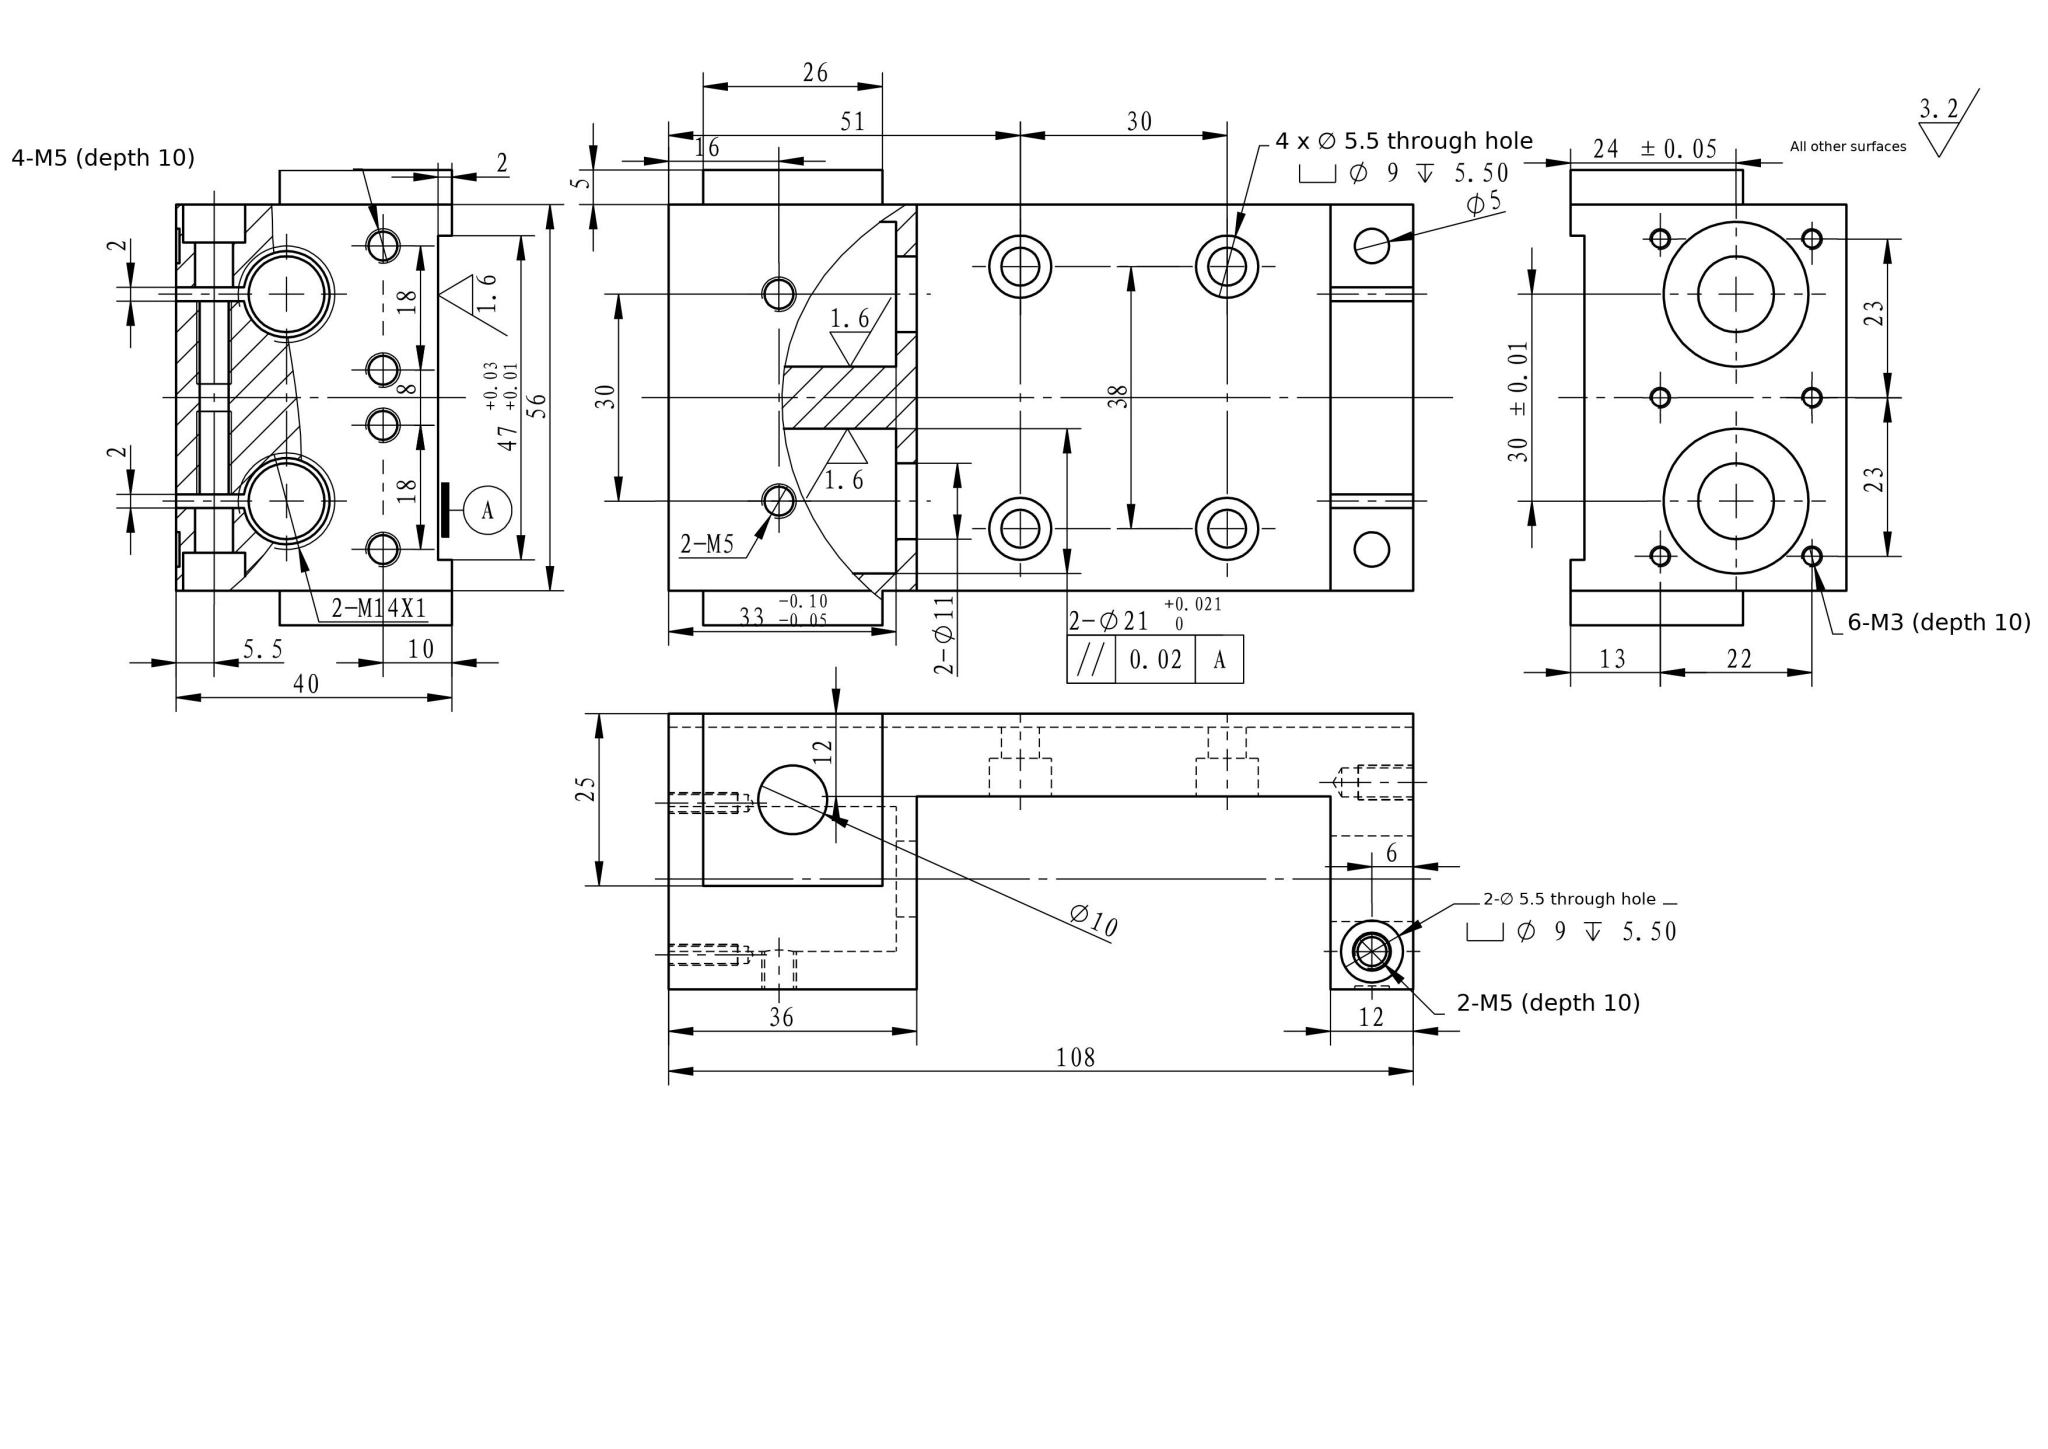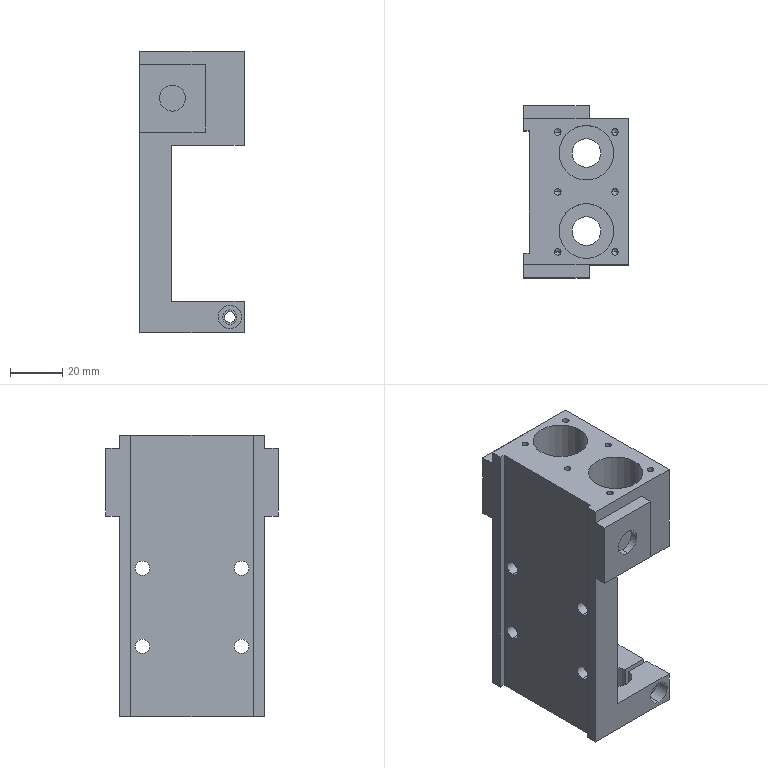Part | SolidWorks | mm | 1 solid | 128 faces | box 40 x 66 x 108 mm | volume 112529 mm3 | cylinder 68 | plane 40 | cone 20 | commonest cylinder face diameters 4.2 x14 2.5 x12 9 x12 5.5 x12 10 x4 5 x4 21 x4 11 x4